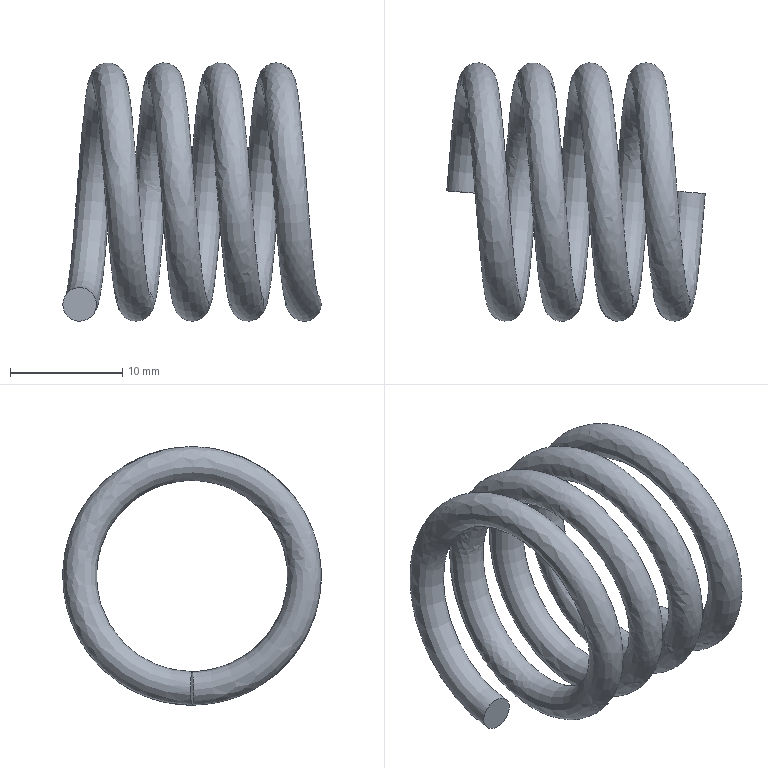Component | NX | SMALL_SPRING | 1 solid | 3 faces | volume 1783 mm3 | plane 2 | spline 1